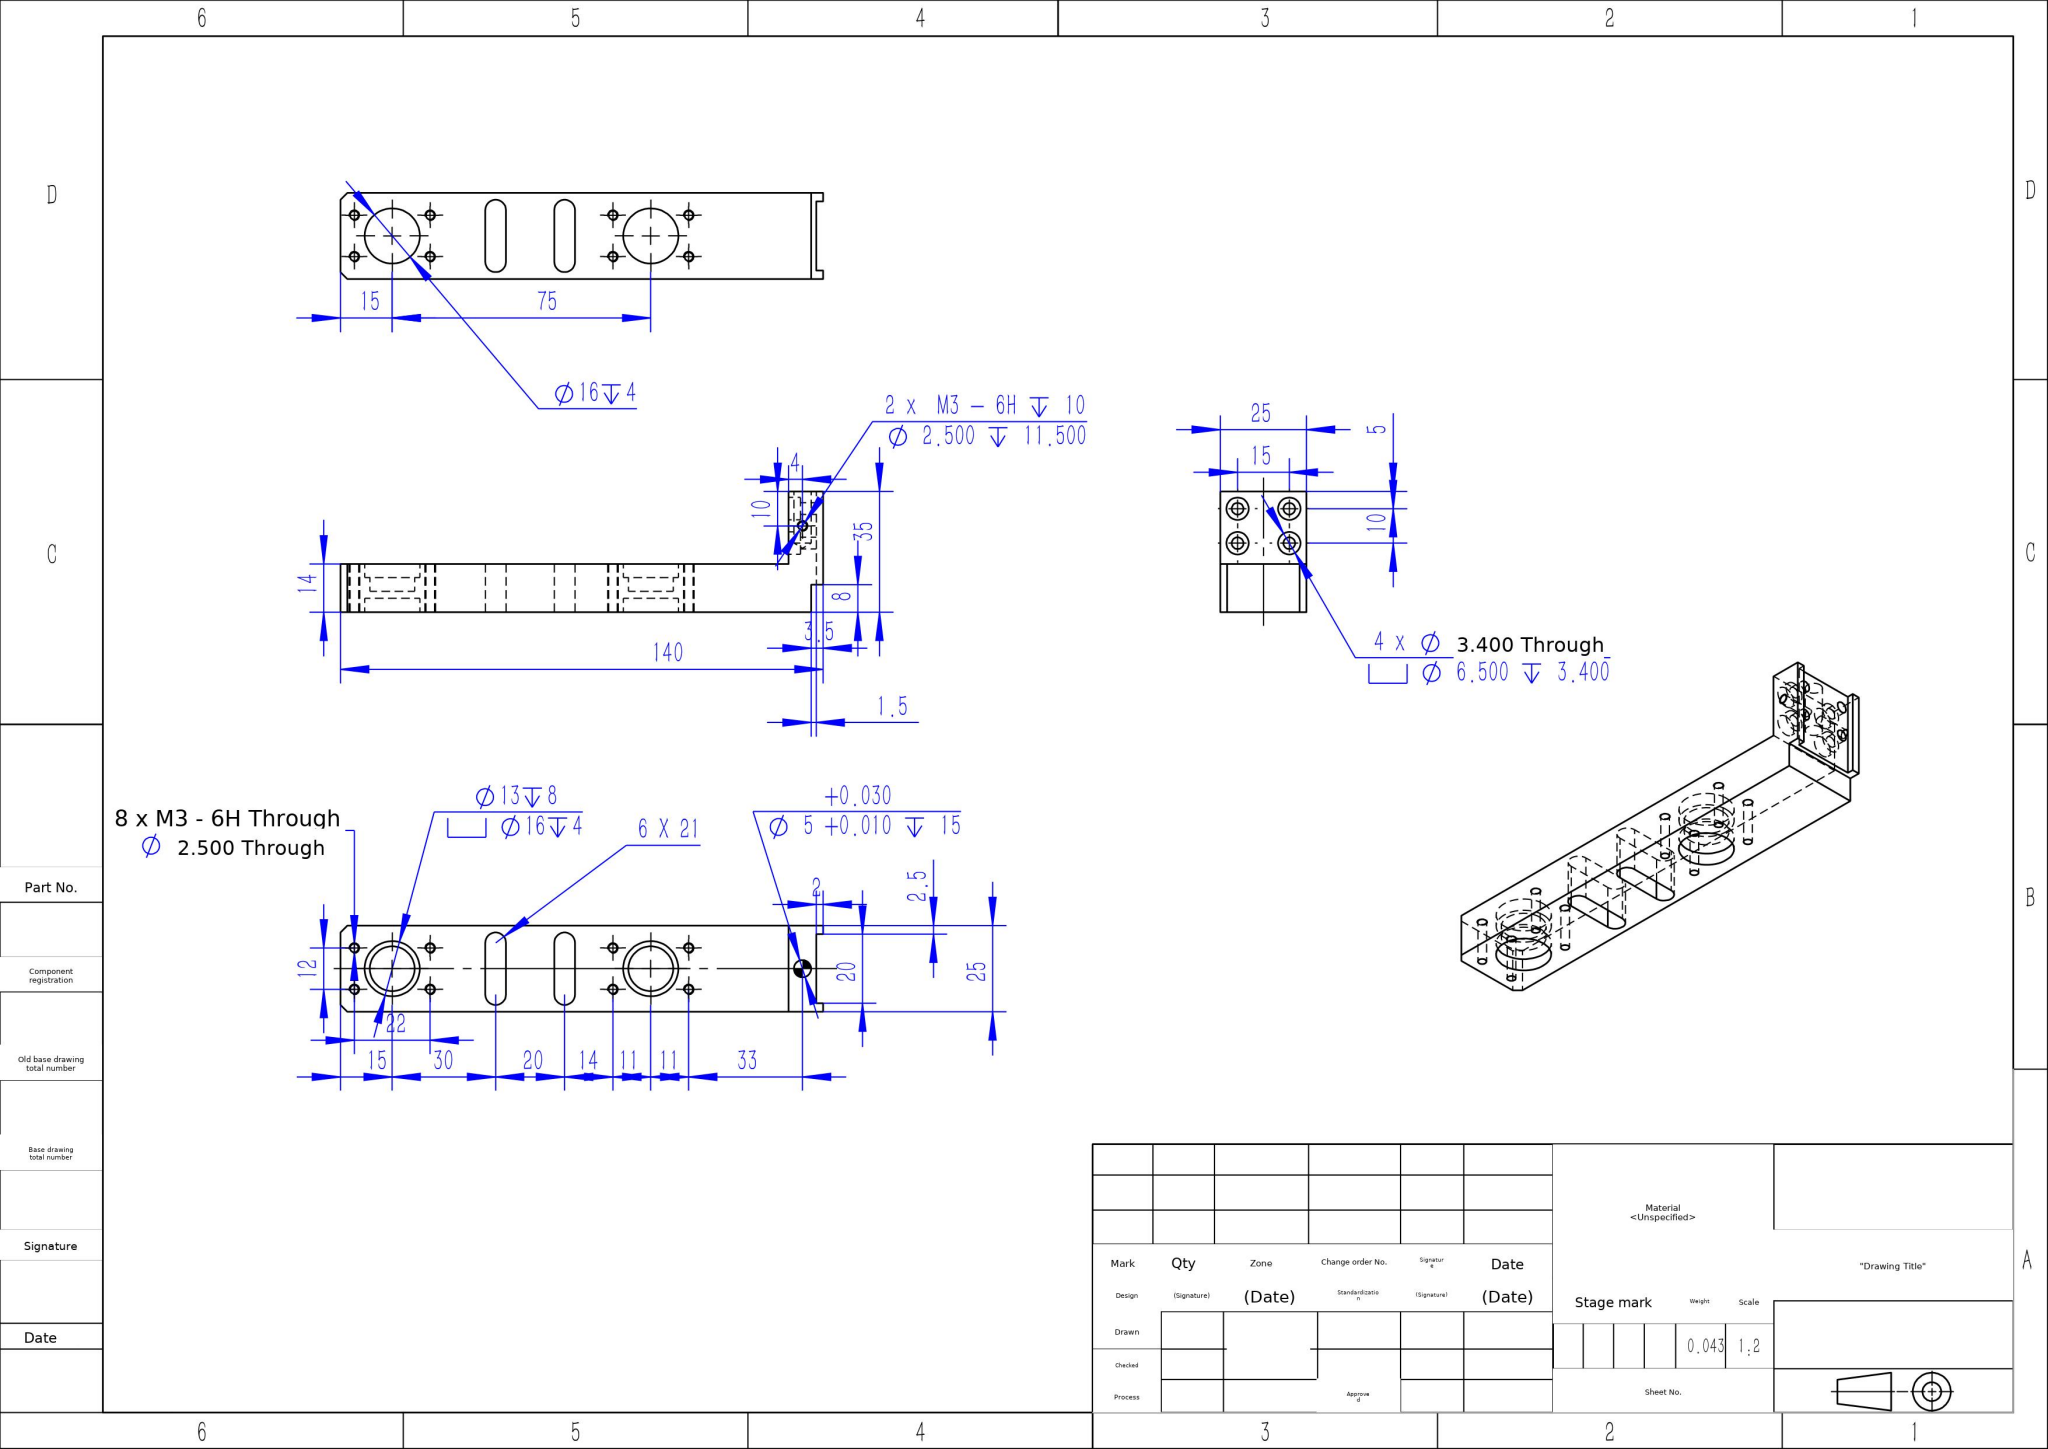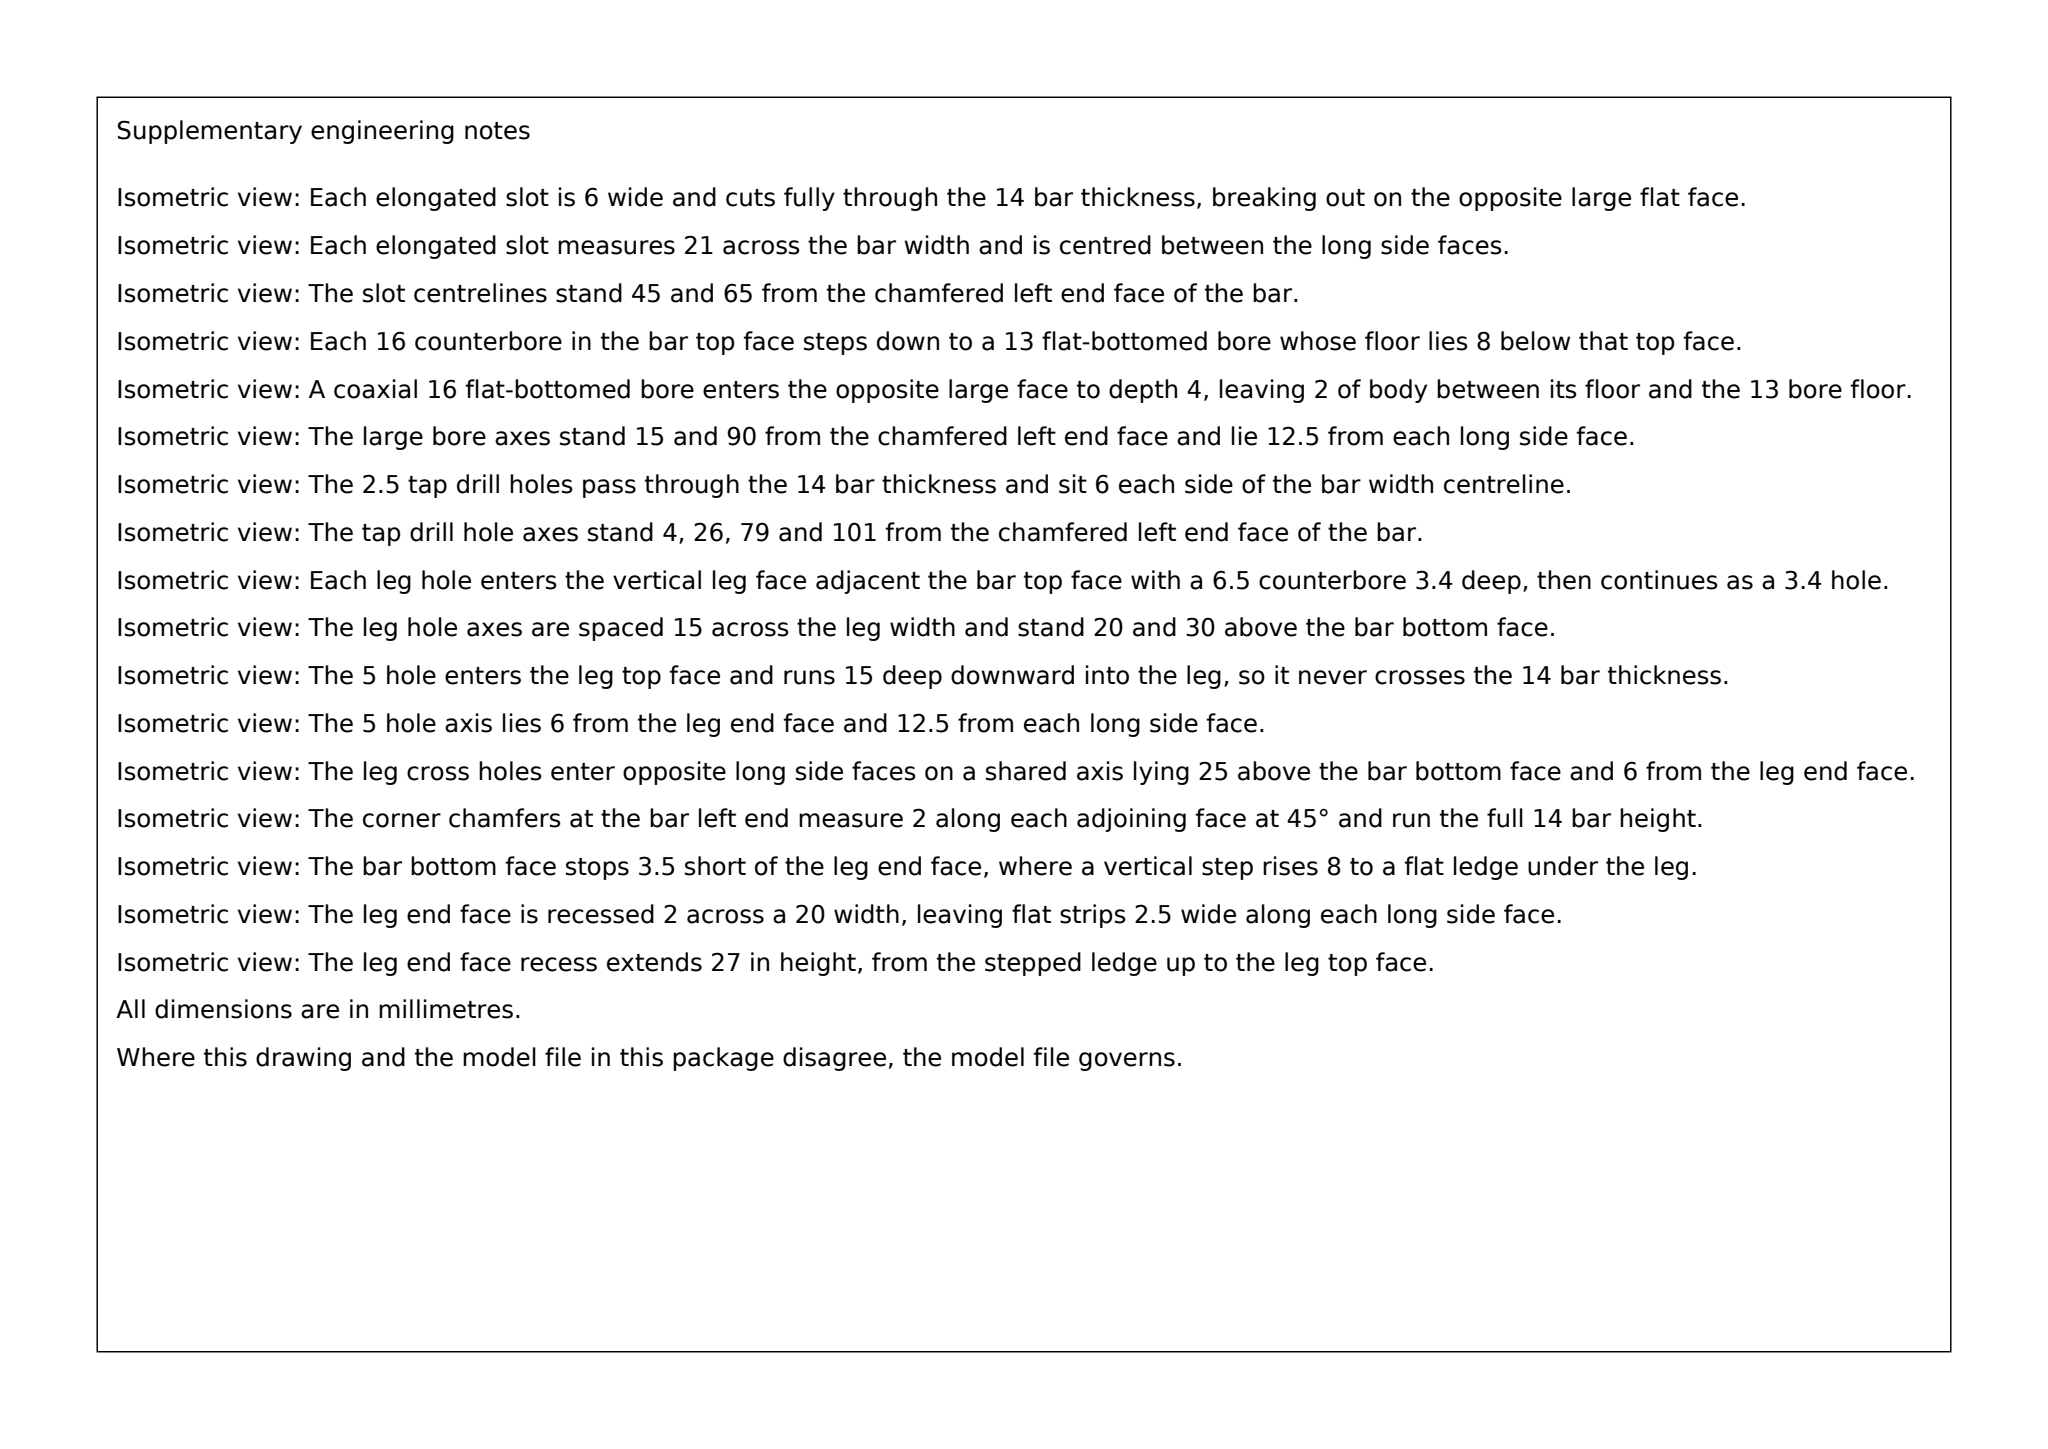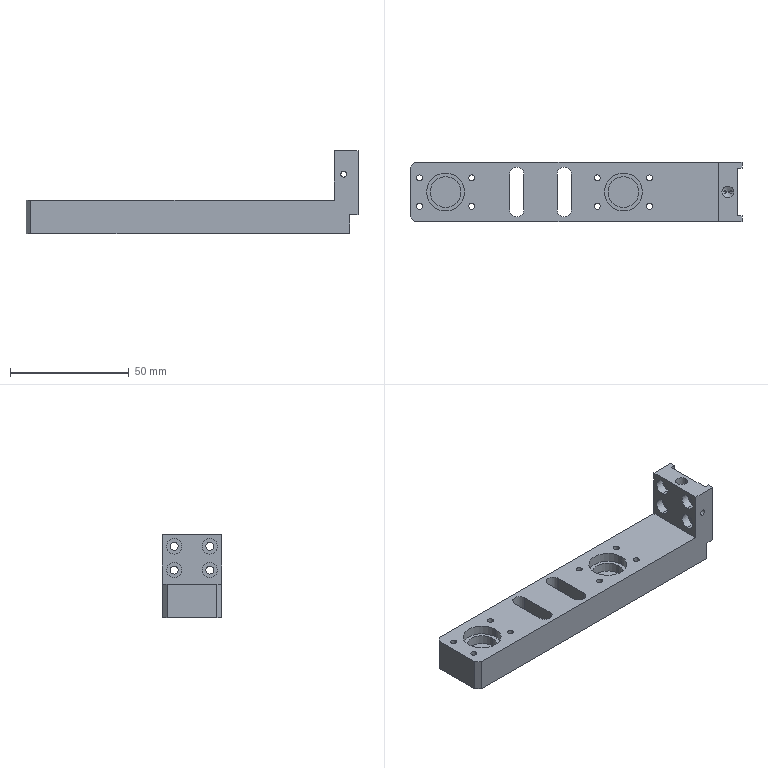Part | SolidWorks | mm | 1 solid | 86 faces | box 140 x 25 x 35 mm | volume 43252 mm3 | cylinder 54 | plane 30 | cone 2 | commonest cylinder face diameters 2.5 x20 16 x8 6.5 x8 3.4 x8 13 x4 6 x4 5 x2
Drawing notes:
Ø13 DP 8 BLIND FROM TOP INCL CBORE Ø16 DP 4; 2ND CBORE Ø16 DP 4 ON BOT FACE | from the solid: Ø16 L4 top cbore z=14-10 and bot cbore z=0-4, Ø13 L4 z=10-6; no thru Ø13
8 X M3-6H THRU: 4 PER BORE ON 22 X 12 PATT, CTRD ON EA Ø13 BORE CL | from the solid: Ø2.5 thru at x=4,26 & 79,101, y=6.5,18.5; Ø13 bores x=15,90 y=12.5 -> ±11 x ±6
2 X M3-6H DP 10: ONE EA FLANGE SIDE FACE, COAXIAL, 6 FROM BACK FACE | from the solid: Ø2.5 y-axis holes x=134 z=25 entering y=0 and y=25 faces; flange faces x=130/140
2X 2 x 2 CHAMFER (45°) ON THE TWO VERTICAL EDGES OF THE FREE END OF THE BAR (X=0 END, AT Y=0 AND Y=25 SIDE FACES), FULL 14 BAR THICKNESS | from the solid: inclined_planes: two 45°/45°/90° faces, size [2.0,2.0,14.0], bbox_from [0,0,0] and [0,23,0]
FLANGE (UPSTAND) THICKNESS 10 FROM INNER FACE (X=130) TO BACK FACE (X=140); CENTRAL BACK FACE RECESSED TO X=138 GIVING 8 THICK OVER Y 2.5 TO 22.5; FLANGE HEIGHT TO Z=35 FROM BAR BOTTOM, BAR THICKNESS 14 | from the solid: axis_planes x=130 (y 0-25, z 14-35), x=138 (y 2.5-22.5, z 8-35), x=140 (y 0-2.5 and 22.5-25, z 8-35), z=35 (x 130-140)
2X M3-6H DP 10 IN FLANGE SIDE FACES (Y=0 AND Y=25), COAXIAL: AXIS AT Z=25 ABOVE BAR BOTTOM FACE (10 BELOW FLANGE TOP) AND X=134 (6 FROM BACK FACE) | from the solid: cylinders: Ø2.5 axis y at [x=134, z=25], from y 0 to 10.3 and y 14.7 to 25
4X Ø3.4 THRU FLANGE WITH CBORE Ø6.5 DP 3.4 MACHINED FROM THE INNER FLANGE FACE X=130 (CBORE X=130 TO 133.4; Ø3.4 RUNS X=133.4 TO RECESSED BACK FACE X=138). HOLE AXES AT Y=5 AND Y=20, Z=20 AND Z=30 FROM BAR BOTTOM | from the solid: cylinders: Ø6.5 axis x from 130 to 133.4 and Ø3.4 axis x from 133.4 to 138, at (y,z)=(5,20),(5,30),(20,20),(20,30); plane x=138 recessed back face
1X Ø5 +0.010/+0.030 DP 15 FROM FLANGE TOP FACE Z=35 (BOTTOM OF HOLE AT Z=20); AXIS AT X=134 (4 FROM INNER FLANGE FACE X=130) AND Y=12.5 (CENTRED ON 25 WIDTH) | from the solid: single cylinder dia 5.0, axis z at (134.0, 12.5), from z=20.0 to z=35.0 (no second Ø5 hole in model)
build123d program:
from build123d import *

# Parameters (mm, degrees)
BOSS_EXTRUDE1_DEPTH                             = 12.5
M3_HEX_SOCKET_HEAD_CAP_SCREW_CBORE2_D           = 3.4
M3_HEX_SOCKET_HEAD_CAP_SCREW_CBORE2_CBORE_D     = 6.5
M3_HEX_SOCKET_HEAD_CAP_SCREW_CBORE2_CBORE_DEPTH = 3.4
SKETCH17_W                                      = 35
SKETCH17_H                                      = 20
CUT_EXTRUDE2_DEPTH                              = 2
SKETCH19_W                                      = 3.5
SKETCH19_H                                      = 8
CUT_EXTRUDE3_DEPTH                              = 147.458
SIZE_MM_DOWEL_PIN_HOLE_1_D                      = 5
SIZE_MM_DOWEL_PIN_HOLE_1_DEPTH                  = 15
SIZE_MM_DOWEL_PIN_HOLE_1_TIP                    = 1.502
CHAMFER1_SIZE                                   = 2
SKETCH27_R                                      = 8
CUT_EXTRUDE4_DEPTH                              = 4
CUT_EXTRUDE5_START                              = -4
SKETCH28_R                                      = 8
CUT_EXTRUDE5_DEPTH                              = 4
SKETCH29_R                                      = 6.5
CUT_EXTRUDE6_DEPTH                              = 4
M3_TAPPED_HOLE2_D                               = 2.5
CUT_EXTRUDE7_DEPTH                              = 143.117


with BuildPart() as part:
    # Sketch1 → Boss-Extrude1 (new, symmetric)
    with BuildSketch(Plane(origin=(0, 0, 0), x_dir=(1, 0, 0), z_dir=(0, 1, 0))):
        Polygon((0, 0), (140, 0), (140, -35), (130, -35), (130, -14), (0, -14), align=None)
    extrude(amount=BOSS_EXTRUDE1_DEPTH, both=True)

    # M3 Hex Socket Head Cap Screw CBORE2 (through all)
    with Locations(Plane.ZY.offset(-130)):
        with Locations((20, 7.5), (30, 7.5), (20, -7.5), (30, -7.5)):
            CounterBoreHole(M3_HEX_SOCKET_HEAD_CAP_SCREW_CBORE2_D / 2, M3_HEX_SOCKET_HEAD_CAP_SCREW_CBORE2_CBORE_D / 2, M3_HEX_SOCKET_HEAD_CAP_SCREW_CBORE2_CBORE_DEPTH)

    # Sketch17 → Cut-Extrude2 (cut)
    with BuildSketch(Plane(origin=(140, 0, 0), x_dir=(0, 0, -1), z_dir=(1, 0, 0))):
        with Locations((-17.5, 0)):
            Rectangle(SKETCH17_W, SKETCH17_H)
    extrude(amount=-CUT_EXTRUDE2_DEPTH, mode=Mode.SUBTRACT)

    # Sketch19 → Cut-Extrude3 (cut, through all)
    with BuildSketch(Plane(origin=(0, 12.5, 0), x_dir=(1, 0, 0), z_dir=(0, 1, 0))):
        with Locations((138.25, -4)):
            Rectangle(SKETCH19_W, SKETCH19_H)
    extrude(amount=-CUT_EXTRUDE3_DEPTH, mode=Mode.SUBTRACT)

    # Size mm Dowel Pin Hole 1
    with Locations(Plane.XY.offset(35)):
        with Locations((134, 0)):
            Hole(SIZE_MM_DOWEL_PIN_HOLE_1_D / 2, depth=SIZE_MM_DOWEL_PIN_HOLE_1_DEPTH)
            with Locations((0, 0, -(SIZE_MM_DOWEL_PIN_HOLE_1_DEPTH + SIZE_MM_DOWEL_PIN_HOLE_1_TIP / 2))):  # 118° drill point
                Cone(0, SIZE_MM_DOWEL_PIN_HOLE_1_D / 2, SIZE_MM_DOWEL_PIN_HOLE_1_TIP, mode=Mode.SUBTRACT)

    # Sketch24 → M3 Tapped Hole1 (revolve, cut)
    with BuildSketch(Plane(origin=(134, 12.5, 25), x_dir=(0, 0, 1), z_dir=(1, 0, 0))):
        Polygon((0, 0), (0, 12.251), (1.25, 11.5), (1.25, 0), align=None)
    m3_tapped_hole1 = revolve(axis=Axis((134, 18.85, 25), (0, -1, 0)), mode=Mode.SUBTRACT)

    # Mirror1: M3 Tapped Hole1 across plane
    add(m3_tapped_hole1.mirror(Plane.ZX), mode=Mode.SUBTRACT)

    # Chamfer1
    chamfer1_edges = [part.edges().sort_by_distance(p)[0] for p in [
        (0, 12.5, 7),
        (0, -12.5, 7),
    ]]
    chamfer(chamfer1_edges, length=CHAMFER1_SIZE)

    # Sketch27 → Cut-Extrude4 (cut)
    with BuildSketch(Plane.XY.offset(14)):
        with Locations((15, 0)):
            Circle(SKETCH27_R)
        with Locations((90, 0)):
            Circle(SKETCH27_R)
    extrude(amount=-CUT_EXTRUDE4_DEPTH, mode=Mode.SUBTRACT)

    # Sketch28 → Cut-Extrude5 (cut)
    with BuildSketch(Plane(origin=(0, 0, 0), x_dir=(-1, 0, 0), z_dir=(0, 0, -1)).offset(CUT_EXTRUDE5_START)):
        with Locations(Location((-15, 0, 0), (0, 0, 180))):
            Circle(SKETCH28_R)
        with Locations(Location((-90, 0, 0), (0, 0, 180))):
            Circle(SKETCH28_R)
    extrude(amount=CUT_EXTRUDE5_DEPTH, mode=Mode.SUBTRACT)

    # Sketch29 → Cut-Extrude6 (cut)
    with BuildSketch(Plane.XY.offset(10)):
        with Locations((15, 0)):
            Circle(SKETCH29_R)
        with Locations((90, 0)):
            Circle(SKETCH29_R)
    extrude(amount=-CUT_EXTRUDE6_DEPTH, mode=Mode.SUBTRACT)

    # M3 Tapped Hole2 (through all)
    with Locations(Plane.XY.offset(14)):
        with Locations((26, 6), (26, -6), (4, 6), (4, -6), (26, -21), (26, -33), (4, -20.205), (4, -33), (26, -48), (26, -60), (4, -48), (4, -60), (101, -48), (101, -60), (79, -60), (79, -48), (101, -33), (101, -21), (79, -33), (79, -21), (101, 6), (101, -6), (79, -6), (79, 6)):
            Hole(M3_TAPPED_HOLE2_D / 2)

    # Sketch32 → Cut-Extrude7 (cut, through all)
    with BuildSketch(Plane.XY.offset(14)):
        with BuildLine():
            Line((48, 7.5), (48, -7.5))
            ThreePointArc((48, -7.5), (45, -10.5), (42, -7.5))
            Line((42, -7.5), (42, 7.5))
            ThreePointArc((42, 7.5), (45, 10.5), (48, 7.5))
        make_face()
        with BuildLine():
            Line((68, 7.5), (68, -7.5))
            ThreePointArc((68, -7.5), (65, -10.5), (62, -7.5))
            Line((62, -7.5), (62, 7.5))
            ThreePointArc((62, 7.5), (65, 10.5), (68, 7.5))
        make_face()
    extrude(amount=-CUT_EXTRUDE7_DEPTH, mode=Mode.SUBTRACT)


solid = part.part